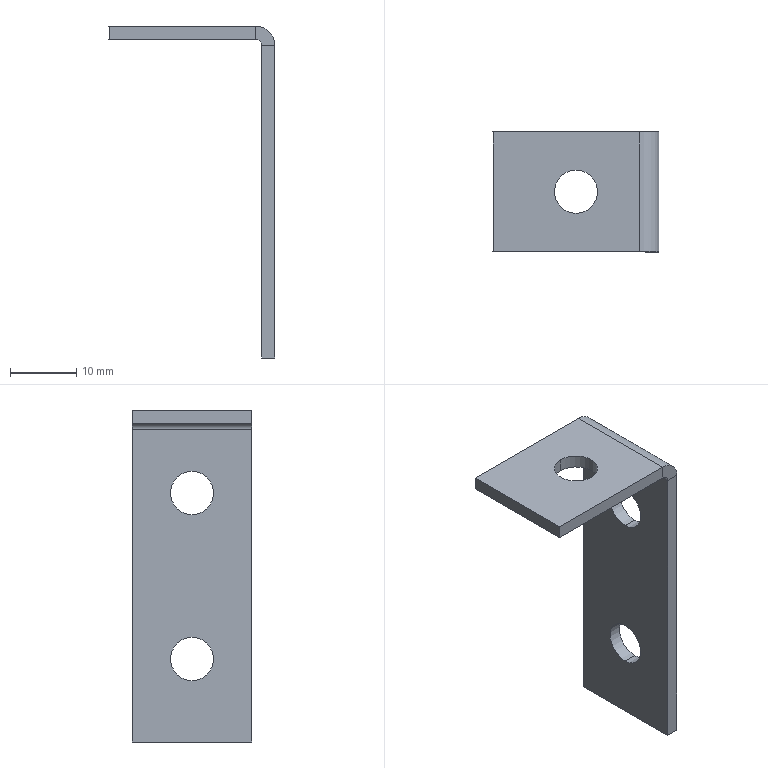Component | SolidWorks | Bracket(No.35)-1 | 1 solid | 20 faces | box 25 x 18 x 50 mm | volume 2398 mm3 | plane 12 | cylinder 8 | commonest cylinder face diameters 6.5 x6 2 x1 6 x1 | material Plain Carbon Steel
STEP:
#1=COLOUR_RGB('',0.7922,0.8196,0.9333);
#2=FILL_AREA_STYLE_COLOUR('',#1);
#3=FILL_AREA_STYLE('',(#2));
#4=SURFACE_STYLE_FILL_AREA(#3);
#5=SURFACE_SIDE_STYLE('',(#4));
#6=SURFACE_STYLE_USAGE(.BOTH.,#5);
#7=PRESENTATION_STYLE_ASSIGNMENT((#6));
#8=CARTESIAN_POINT('',(13.287,15.128,-2.047));
#9=VERTEX_POINT('',#8);
#10=CARTESIAN_POINT('',(13.287,15.384,-2.047));
#11=VERTEX_POINT('',#10);
#12=CARTESIAN_POINT('',(13.287,15.256,-2.047));
#13=DIRECTION('',(0.,-0.,1.));
#14=DIRECTION('',(0.,1.,0.));
#15=AXIS2_PLACEMENT_3D('',#12,#13,#14);
#16=CIRCLE('',#15,0.128);
#17=EDGE_CURVE('',#9,#11,#16,.T.);
#18=ORIENTED_EDGE('',*,*,#17,.F.);
#19=CARTESIAN_POINT('',(13.287,15.128,-1.969));
#20=VERTEX_POINT('',#19);
#21=CARTESIAN_POINT('',(13.287,15.128,-2.047));
#22=DIRECTION('',(0.,-0.,1.));
#23=VECTOR('',#22,39.37);
#24=LINE('',#21,#23);
#25=EDGE_CURVE('',#9,#20,#24,.T.);
#26=ORIENTED_EDGE('',*,*,#25,.T.);
#27=CARTESIAN_POINT('',(13.287,15.384,-1.969));
#28=VERTEX_POINT('',#27);
#29=CARTESIAN_POINT('',(13.287,15.256,-1.969));
#30=DIRECTION('',(0.,-0.,1.));
#31=DIRECTION('',(0.,1.,0.));
#32=AXIS2_PLACEMENT_3D('',#29,#30,#31);
#33=CIRCLE('',#32,0.128);
#34=EDGE_CURVE('',#20,#28,#33,.T.);
#35=ORIENTED_EDGE('',*,*,#34,.T.);
#36=CARTESIAN_POINT('',(13.287,15.384,-2.047));
#37=DIRECTION('',(0.,-0.,1.));
#38=VECTOR('',#37,39.37);
#39=LINE('',#36,#38);
#40=EDGE_CURVE('',#11,#28,#39,.T.);
#41=ORIENTED_EDGE('',*,*,#40,.F.);
#42=EDGE_LOOP('',(#18,#26,#35,#41));
#43=FACE_OUTER_BOUND('',#42,.T.);
#44=CARTESIAN_POINT('',(13.287,15.256,-2.047));
#45=DIRECTION('',(0.,-0.,1.));
#46=DIRECTION('',(0.,1.,0.));
#47=AXIS2_PLACEMENT_3D('',#44,#45,#46);
#48=CYLINDRICAL_SURFACE('',#47,0.128);
#49=ADVANCED_FACE('',(#43),#48,.F.);
#50=CARTESIAN_POINT('',(13.78,15.256,-2.333));
#51=VERTEX_POINT('',#50);
#52=CARTESIAN_POINT('',(13.78,15.256,-2.589));
#53=VERTEX_POINT('',#52);
#54=CARTESIAN_POINT('',(13.78,15.256,-2.461));
#55=DIRECTION('',(-1.,-0.,-0.));
#56=DIRECTION('',(0.,0.,-1.));
#57=AXIS2_PLACEMENT_3D('',#54,#55,#56);
#58=CIRCLE('',#57,0.128);
#59=EDGE_CURVE('',#51,#53,#58,.T.);
#60=ORIENTED_EDGE('',*,*,#59,.F.);
#61=CARTESIAN_POINT('',(13.701,15.256,-2.333));
#62=VERTEX_POINT('',#61);
#63=CARTESIAN_POINT('',(13.78,15.256,-2.333));
#64=DIRECTION('',(-1.,-0.,-0.));
#65=VECTOR('',#64,39.37);
#66=LINE('',#63,#65);
#67=EDGE_CURVE('',#51,#62,#66,.T.);
#68=ORIENTED_EDGE('',*,*,#67,.T.);
#69=CARTESIAN_POINT('',(13.701,15.256,-2.589));
#70=VERTEX_POINT('',#69);
#71=CARTESIAN_POINT('',(13.701,15.256,-2.461));
#72=DIRECTION('',(-1.,-0.,-0.));
#73=DIRECTION('',(0.,0.,-1.));
#74=AXIS2_PLACEMENT_3D('',#71,#72,#73);
#75=CIRCLE('',#74,0.128);
#76=EDGE_CURVE('',#62,#70,#75,.T.);
#77=ORIENTED_EDGE('',*,*,#76,.T.);
#78=CARTESIAN_POINT('',(13.78,15.256,-2.589));
#79=DIRECTION('',(-1.,-0.,-0.));
#80=VECTOR('',#79,39.37);
#81=LINE('',#78,#80);
#82=EDGE_CURVE('',#53,#70,#81,.T.);
#83=ORIENTED_EDGE('',*,*,#82,.F.);
#84=EDGE_LOOP('',(#60,#68,#77,#83));
#85=FACE_OUTER_BOUND('',#84,.T.);
#86=CARTESIAN_POINT('',(13.78,15.256,-2.461));
#87=DIRECTION('',(-1.,-0.,-0.));
#88=DIRECTION('',(0.,0.,-1.));
#89=AXIS2_PLACEMENT_3D('',#86,#87,#88);
#90=CYLINDRICAL_SURFACE('',#89,0.128);
#91=ADVANCED_FACE('',(#85),#90,.F.);
#92=CARTESIAN_POINT('',(13.78,15.256,-3.317));
#93=VERTEX_POINT('',#92);
#94=CARTESIAN_POINT('',(13.78,15.256,-3.573));
#95=VERTEX_POINT('',#94);
#96=CARTESIAN_POINT('',(13.78,15.256,-3.445));
#97=DIRECTION('',(-1.,-0.,-0.));
#98=DIRECTION('',(0.,0.,-1.));
#99=AXIS2_PLACEMENT_3D('',#96,#97,#98);
#100=CIRCLE('',#99,0.128);
#101=EDGE_CURVE('',#93,#95,#100,.T.);
#102=ORIENTED_EDGE('',*,*,#101,.F.);
#103=CARTESIAN_POINT('',(13.701,15.256,-3.317));
#104=VERTEX_POINT('',#103);
#105=CARTESIAN_POINT('',(13.78,15.256,-3.317));
#106=DIRECTION('',(-1.,-0.,-0.));
#107=VECTOR('',#106,39.37);
#108=LINE('',#105,#107);
#109=EDGE_CURVE('',#93,#104,#108,.T.);
#110=ORIENTED_EDGE('',*,*,#109,.T.);
#111=CARTESIAN_POINT('',(13.701,15.256,-3.573));
#112=VERTEX_POINT('',#111);
#113=CARTESIAN_POINT('',(13.701,15.256,-3.445));
#114=DIRECTION('',(-1.,-0.,-0.));
#115=DIRECTION('',(0.,0.,-1.));
#116=AXIS2_PLACEMENT_3D('',#113,#114,#115);
#117=CIRCLE('',#116,0.128);
#118=EDGE_CURVE('',#104,#112,#117,.T.);
#119=ORIENTED_EDGE('',*,*,#118,.T.);
#120=CARTESIAN_POINT('',(13.78,15.256,-3.573));
#121=DIRECTION('',(-1.,-0.,-0.));
#122=VECTOR('',#121,39.37);
#123=LINE('',#120,#122);
#124=EDGE_CURVE('',#95,#112,#123,.T.);
#125=ORIENTED_EDGE('',*,*,#124,.F.);
#126=EDGE_LOOP('',(#102,#110,#119,#125));
#127=FACE_OUTER_BOUND('',#126,.T.);
#128=CARTESIAN_POINT('',(13.78,15.256,-3.445));
#129=DIRECTION('',(-1.,-0.,-0.));
#130=DIRECTION('',(0.,0.,-1.));
#131=AXIS2_PLACEMENT_3D('',#128,#129,#130);
#132=CYLINDRICAL_SURFACE('',#131,0.128);
#133=ADVANCED_FACE('',(#127),#132,.F.);
#134=CARTESIAN_POINT('',(13.78,14.902,-2.087));
#135=VERTEX_POINT('',#134);
#136=CARTESIAN_POINT('',(13.701,14.902,-2.087));
#137=VERTEX_POINT('',#136);
#138=CARTESIAN_POINT('',(13.78,14.902,-2.087));
#139=DIRECTION('',(-1.,-0.,0.));
#140=VECTOR('',#139,39.37);
#141=LINE('',#138,#140);
#142=EDGE_CURVE('',#135,#137,#141,.T.);
#143=ORIENTED_EDGE('',*,*,#142,.F.);
#144=CARTESIAN_POINT('',(13.661,14.902,-1.969));
#145=VERTEX_POINT('',#144);
#146=CARTESIAN_POINT('',(13.661,14.902,-2.087));
#147=DIRECTION('',(0.,-1.,-0.));
#148=DIRECTION('',(1.,0.,0.));
#149=AXIS2_PLACEMENT_3D('',#146,#147,#148);
#150=CIRCLE('',#149,0.1181);
#151=EDGE_CURVE('',#135,#145,#150,.T.);
#152=ORIENTED_EDGE('',*,*,#151,.T.);
#153=CARTESIAN_POINT('',(13.661,14.902,-2.047));
#154=VERTEX_POINT('',#153);
#155=CARTESIAN_POINT('',(13.661,14.902,-2.047));
#156=DIRECTION('',(0.,-0.,1.));
#157=VECTOR('',#156,39.37);
#158=LINE('',#155,#157);
#159=EDGE_CURVE('',#154,#145,#158,.T.);
#160=ORIENTED_EDGE('',*,*,#159,.F.);
#161=CARTESIAN_POINT('',(13.661,14.902,-2.087));
#162=DIRECTION('',(0.,-1.,-0.));
#163=DIRECTION('',(-1.,0.,0.));
#164=AXIS2_PLACEMENT_3D('',#161,#162,#163);
#165=CIRCLE('',#164,0.03937);
#166=EDGE_CURVE('',#137,#154,#165,.T.);
#167=ORIENTED_EDGE('',*,*,#166,.F.);
#168=EDGE_LOOP('',(#143,#152,#160,#167));
#169=FACE_OUTER_BOUND('',#168,.T.);
#170=CARTESIAN_POINT('',(13.78,14.902,-2.087));
#171=DIRECTION('',(0.,-1.,-0.));
#172=DIRECTION('',(-1.,-0.,0.));
#173=AXIS2_PLACEMENT_3D('',#170,#171,#172);
#174=PLANE('',#173);
#175=ADVANCED_FACE('',(#169),#174,.T.);
#176=CARTESIAN_POINT('',(13.78,14.902,-3.937));
#177=VERTEX_POINT('',#176);
#178=CARTESIAN_POINT('',(13.78,14.902,-3.937));
#179=DIRECTION('',(-0.,-0.,1.));
#180=VECTOR('',#179,39.37);
#181=LINE('',#178,#180);
#182=EDGE_CURVE('',#177,#135,#181,.T.);
#183=ORIENTED_EDGE('',*,*,#182,.T.);
#184=ORIENTED_EDGE('',*,*,#142,.T.);
#185=CARTESIAN_POINT('',(13.701,14.902,-3.937));
#186=VERTEX_POINT('',#185);
#187=CARTESIAN_POINT('',(13.701,14.902,-3.937));
#188=DIRECTION('',(-0.,-0.,1.));
#189=VECTOR('',#188,39.37);
#190=LINE('',#187,#189);
#191=EDGE_CURVE('',#186,#137,#190,.T.);
#192=ORIENTED_EDGE('',*,*,#191,.F.);
#193=CARTESIAN_POINT('',(13.78,14.902,-3.937));
#194=DIRECTION('',(-1.,-0.,0.));
#195=VECTOR('',#194,39.37);
#196=LINE('',#193,#195);
#197=EDGE_CURVE('',#177,#186,#196,.T.);
#198=ORIENTED_EDGE('',*,*,#197,.F.);
#199=EDGE_LOOP('',(#183,#184,#192,#198));
#200=FACE_OUTER_BOUND('',#199,.T.);
#201=CARTESIAN_POINT('',(13.661,14.902,-2.047));
#202=DIRECTION('',(0.,-1.,-0.));
#203=DIRECTION('',(-1.,-0.,0.));
#204=AXIS2_PLACEMENT_3D('',#201,#202,#203);
#205=PLANE('',#204);
#206=ADVANCED_FACE('',(#200),#205,.T.);
#207=CARTESIAN_POINT('',(13.661,15.61,-1.969));
#208=VERTEX_POINT('',#207);
#209=CARTESIAN_POINT('',(13.661,15.61,-2.047));
#210=VERTEX_POINT('',#209);
#211=CARTESIAN_POINT('',(13.661,15.61,-1.969));
#212=DIRECTION('',(-0.,0.,-1.));
#213=VECTOR('',#212,39.37);
#214=LINE('',#211,#213);
#215=EDGE_CURVE('',#208,#210,#214,.T.);
#216=ORIENTED_EDGE('',*,*,#215,.F.);
#217=CARTESIAN_POINT('',(13.78,15.61,-2.087));
#218=VERTEX_POINT('',#217);
#219=CARTESIAN_POINT('',(13.661,15.61,-2.087));
#220=DIRECTION('',(0.,-1.,-0.));
#221=DIRECTION('',(1.,0.,0.));
#222=AXIS2_PLACEMENT_3D('',#219,#220,#221);
#223=CIRCLE('',#222,0.1181);
#224=EDGE_CURVE('',#218,#208,#223,.T.);
#225=ORIENTED_EDGE('',*,*,#224,.F.);
#226=CARTESIAN_POINT('',(13.701,15.61,-2.087));
#227=VERTEX_POINT('',#226);
#228=CARTESIAN_POINT('',(13.701,15.61,-2.087));
#229=DIRECTION('',(1.,0.,-0.));
#230=VECTOR('',#229,39.37);
#231=LINE('',#228,#230);
#232=EDGE_CURVE('',#227,#218,#231,.T.);
#233=ORIENTED_EDGE('',*,*,#232,.F.);
#234=CARTESIAN_POINT('',(13.661,15.61,-2.087));
#235=DIRECTION('',(0.,-1.,-0.));
#236=DIRECTION('',(-1.,0.,0.));
#237=AXIS2_PLACEMENT_3D('',#234,#235,#236);
#238=CIRCLE('',#237,0.03937);
#239=EDGE_CURVE('',#227,#210,#238,.T.);
#240=ORIENTED_EDGE('',*,*,#239,.T.);
#241=EDGE_LOOP('',(#216,#225,#233,#240));
#242=FACE_OUTER_BOUND('',#241,.T.);
#243=CARTESIAN_POINT('',(13.661,15.61,-1.969));
#244=DIRECTION('',(-0.,1.,0.));
#245=DIRECTION('',(1.,0.,-0.));
#246=AXIS2_PLACEMENT_3D('',#243,#244,#245);
#247=PLANE('',#246);
#248=ADVANCED_FACE('',(#242),#247,.T.);
#249=CARTESIAN_POINT('',(12.795,15.61,-1.969));
#250=VERTEX_POINT('',#249);
#251=CARTESIAN_POINT('',(13.78,15.61,-1.969));
#252=DIRECTION('',(-1.,-0.,0.));
#253=VECTOR('',#252,39.37);
#254=LINE('',#251,#253);
#255=EDGE_CURVE('',#208,#250,#254,.T.);
#256=ORIENTED_EDGE('',*,*,#255,.F.);
#257=ORIENTED_EDGE('',*,*,#215,.T.);
#258=CARTESIAN_POINT('',(12.795,15.61,-2.047));
#259=VERTEX_POINT('',#258);
#260=CARTESIAN_POINT('',(13.78,15.61,-2.047));
#261=DIRECTION('',(-1.,-0.,0.));
#262=VECTOR('',#261,39.37);
#263=LINE('',#260,#262);
#264=EDGE_CURVE('',#210,#259,#263,.T.);
#265=ORIENTED_EDGE('',*,*,#264,.T.);
#266=CARTESIAN_POINT('',(12.795,15.61,-2.047));
#267=DIRECTION('',(0.,-0.,1.));
#268=VECTOR('',#267,39.37);
#269=LINE('',#266,#268);
#270=EDGE_CURVE('',#259,#250,#269,.T.);
#271=ORIENTED_EDGE('',*,*,#270,.T.);
#272=EDGE_LOOP('',(#256,#257,#265,#271));
#273=FACE_OUTER_BOUND('',#272,.T.);
#274=CARTESIAN_POINT('',(13.701,15.61,-2.087));
#275=DIRECTION('',(-0.,1.,0.));
#276=DIRECTION('',(1.,0.,-0.));
#277=AXIS2_PLACEMENT_3D('',#274,#275,#276);
#278=PLANE('',#277);
#279=ADVANCED_FACE('',(#273),#278,.T.);
#280=CARTESIAN_POINT('',(13.287,15.256,-1.969));
#281=DIRECTION('',(0.,-0.,1.));
#282=DIRECTION('',(0.,1.,0.));
#283=AXIS2_PLACEMENT_3D('',#280,#281,#282);
#284=CIRCLE('',#283,0.128);
#285=EDGE_CURVE('',#28,#20,#284,.T.);
#286=ORIENTED_EDGE('',*,*,#285,.F.);
#287=ORIENTED_EDGE('',*,*,#34,.F.);
#288=EDGE_LOOP('',(#286,#287));
#289=FACE_BOUND('',#288,.T.);
#290=ORIENTED_EDGE('',*,*,#255,.T.);
#291=CARTESIAN_POINT('',(12.795,14.902,-1.969));
#292=VERTEX_POINT('',#291);
#293=CARTESIAN_POINT('',(12.795,14.902,-1.969));
#294=DIRECTION('',(-0.,1.,0.));
#295=VECTOR('',#294,39.37);
#296=LINE('',#293,#295);
#297=EDGE_CURVE('',#292,#250,#296,.T.);
#298=ORIENTED_EDGE('',*,*,#297,.F.);
#299=CARTESIAN_POINT('',(13.78,14.902,-1.969));
#300=DIRECTION('',(-1.,-0.,0.));
#301=VECTOR('',#300,39.37);
#302=LINE('',#299,#301);
#303=EDGE_CURVE('',#145,#292,#302,.T.);
#304=ORIENTED_EDGE('',*,*,#303,.F.);
#305=CARTESIAN_POINT('',(13.661,14.902,-1.969));
#306=DIRECTION('',(-0.,1.,0.));
#307=VECTOR('',#306,39.37);
#308=LINE('',#305,#307);
#309=EDGE_CURVE('',#145,#208,#308,.T.);
#310=ORIENTED_EDGE('',*,*,#309,.T.);
#311=EDGE_LOOP('',(#290,#298,#304,#310));
#312=FACE_OUTER_BOUND('',#311,.T.);
#313=CARTESIAN_POINT('',(13.78,14.902,-1.969));
#314=DIRECTION('',(-0.,0.,-1.));
#315=DIRECTION('',(0.,-1.,-0.));
#316=AXIS2_PLACEMENT_3D('',#313,#314,#315);
#317=PLANE('',#316);
#318=ADVANCED_FACE('',(#289,#312),#317,.F.);
#319=ORIENTED_EDGE('',*,*,#270,.F.);
#320=CARTESIAN_POINT('',(12.795,14.902,-2.047));
#321=VERTEX_POINT('',#320);
#322=CARTESIAN_POINT('',(12.795,14.902,-2.047));
#323=DIRECTION('',(-0.,1.,0.));
#324=VECTOR('',#323,39.37);
#325=LINE('',#322,#324);
#326=EDGE_CURVE('',#321,#259,#325,.T.);
#327=ORIENTED_EDGE('',*,*,#326,.F.);
#328=CARTESIAN_POINT('',(12.795,14.902,-2.047));
#329=DIRECTION('',(0.,-0.,1.));
#330=VECTOR('',#329,39.37);
#331=LINE('',#328,#330);
#332=EDGE_CURVE('',#321,#292,#331,.T.);
#333=ORIENTED_EDGE('',*,*,#332,.T.);
#334=ORIENTED_EDGE('',*,*,#297,.T.);
#335=EDGE_LOOP('',(#319,#327,#333,#334));
#336=FACE_OUTER_BOUND('',#335,.T.);
#337=CARTESIAN_POINT('',(12.795,14.902,-2.047));
#338=DIRECTION('',(-1.,-0.,0.));
#339=DIRECTION('',(-0.,1.,0.));
#340=AXIS2_PLACEMENT_3D('',#337,#338,#339);
#341=PLANE('',#340);
#342=ADVANCED_FACE('',(#336),#341,.T.);
#343=CARTESIAN_POINT('',(13.287,15.256,-2.047));
#344=DIRECTION('',(0.,-0.,1.));
#345=DIRECTION('',(0.,1.,0.));
#346=AXIS2_PLACEMENT_3D('',#343,#344,#345);
#347=CIRCLE('',#346,0.128);
#348=EDGE_CURVE('',#11,#9,#347,.T.);
#349=ORIENTED_EDGE('',*,*,#348,.T.);
#350=ORIENTED_EDGE('',*,*,#17,.T.);
#351=EDGE_LOOP('',(#349,#350));
#352=FACE_BOUND('',#351,.T.);
#353=ORIENTED_EDGE('',*,*,#264,.F.);
#354=CARTESIAN_POINT('',(13.661,14.902,-2.047));
#355=DIRECTION('',(-0.,1.,0.));
#356=VECTOR('',#355,39.37);
#357=LINE('',#354,#356);
#358=EDGE_CURVE('',#154,#210,#357,.T.);
#359=ORIENTED_EDGE('',*,*,#358,.F.);
#360=CARTESIAN_POINT('',(13.78,14.902,-2.047));
#361=DIRECTION('',(-1.,-0.,0.));
#362=VECTOR('',#361,39.37);
#363=LINE('',#360,#362);
#364=EDGE_CURVE('',#154,#321,#363,.T.);
#365=ORIENTED_EDGE('',*,*,#364,.T.);
#366=ORIENTED_EDGE('',*,*,#326,.T.);
#367=EDGE_LOOP('',(#353,#359,#365,#366));
#368=FACE_OUTER_BOUND('',#367,.T.);
#369=CARTESIAN_POINT('',(13.78,14.902,-2.047));
#370=DIRECTION('',(-0.,0.,-1.));
#371=DIRECTION('',(0.,-1.,-0.));
#372=AXIS2_PLACEMENT_3D('',#369,#370,#371);
#373=PLANE('',#372);
#374=ADVANCED_FACE('',(#352,#368),#373,.T.);
#375=ORIENTED_EDGE('',*,*,#239,.F.);
#376=CARTESIAN_POINT('',(13.701,14.902,-2.087));
#377=DIRECTION('',(-0.,1.,0.));
#378=VECTOR('',#377,39.37);
#379=LINE('',#376,#378);
#380=EDGE_CURVE('',#137,#227,#379,.T.);
#381=ORIENTED_EDGE('',*,*,#380,.F.);
#382=ORIENTED_EDGE('',*,*,#166,.T.);
#383=ORIENTED_EDGE('',*,*,#358,.T.);
#384=EDGE_LOOP('',(#375,#381,#382,#383));
#385=FACE_OUTER_BOUND('',#384,.T.);
#386=CARTESIAN_POINT('',(13.661,14.902,-2.087));
#387=DIRECTION('',(-0.,1.,0.));
#388=DIRECTION('',(1.,0.,0.));
#389=AXIS2_PLACEMENT_3D('',#386,#387,#388);
#390=CYLINDRICAL_SURFACE('',#389,0.03937);
#391=ADVANCED_FACE('',(#385),#390,.F.);
#392=CARTESIAN_POINT('',(13.701,15.256,-2.461));
#393=DIRECTION('',(-1.,-0.,-0.));
#394=DIRECTION('',(0.,0.,-1.));
#395=AXIS2_PLACEMENT_3D('',#392,#393,#394);
#396=CIRCLE('',#395,0.128);
#397=EDGE_CURVE('',#70,#62,#396,.T.);
#398=ORIENTED_EDGE('',*,*,#397,.F.);
#399=ORIENTED_EDGE('',*,*,#76,.F.);
#400=EDGE_LOOP('',(#398,#399));
#401=FACE_BOUND('',#400,.T.);
#402=CARTESIAN_POINT('',(13.701,15.256,-3.445));
#403=DIRECTION('',(-1.,-0.,-0.));
#404=DIRECTION('',(0.,0.,-1.));
#405=AXIS2_PLACEMENT_3D('',#402,#403,#404);
#406=CIRCLE('',#405,0.128);
#407=EDGE_CURVE('',#112,#104,#406,.T.);
#408=ORIENTED_EDGE('',*,*,#407,.F.);
#409=ORIENTED_EDGE('',*,*,#118,.F.);
#410=EDGE_LOOP('',(#408,#409));
#411=FACE_BOUND('',#410,.T.);
#412=CARTESIAN_POINT('',(13.701,15.61,-3.937));
#413=VERTEX_POINT('',#412);
#414=CARTESIAN_POINT('',(13.701,15.61,-3.937));
#415=DIRECTION('',(-0.,-0.,1.));
#416=VECTOR('',#415,39.37);
#417=LINE('',#414,#416);
#418=EDGE_CURVE('',#413,#227,#417,.T.);
#419=ORIENTED_EDGE('',*,*,#418,.F.);
#420=CARTESIAN_POINT('',(13.701,14.902,-3.937));
#421=DIRECTION('',(-0.,1.,0.));
#422=VECTOR('',#421,39.37);
#423=LINE('',#420,#422);
#424=EDGE_CURVE('',#186,#413,#423,.T.);
#425=ORIENTED_EDGE('',*,*,#424,.F.);
#426=ORIENTED_EDGE('',*,*,#191,.T.);
#427=ORIENTED_EDGE('',*,*,#380,.T.);
#428=EDGE_LOOP('',(#419,#425,#426,#427));
#429=FACE_OUTER_BOUND('',#428,.T.);
#430=CARTESIAN_POINT('',(13.701,14.902,-3.937));
#431=DIRECTION('',(-1.,-0.,-0.));
#432=DIRECTION('',(0.,0.,-1.));
#433=AXIS2_PLACEMENT_3D('',#430,#431,#432);
#434=PLANE('',#433);
#435=ADVANCED_FACE('',(#401,#411,#429),#434,.T.);
#436=CARTESIAN_POINT('',(13.78,15.61,-3.937));
#437=VERTEX_POINT('',#436);
#438=CARTESIAN_POINT('',(13.78,15.61,-3.937));
#439=DIRECTION('',(-1.,-0.,0.));
#440=VECTOR('',#439,39.37);
#441=LINE('',#438,#440);
#442=EDGE_CURVE('',#437,#413,#441,.T.);
#443=ORIENTED_EDGE('',*,*,#442,.F.);
#444=CARTESIAN_POINT('',(13.78,14.902,-3.937));
#445=DIRECTION('',(-0.,1.,0.));
#446=VECTOR('',#445,39.37);
#447=LINE('',#444,#446);
#448=EDGE_CURVE('',#177,#437,#447,.T.);
#449=ORIENTED_EDGE('',*,*,#448,.F.);
#450=ORIENTED_EDGE('',*,*,#197,.T.);
#451=ORIENTED_EDGE('',*,*,#424,.T.);
#452=EDGE_LOOP('',(#443,#449,#450,#451));
#453=FACE_OUTER_BOUND('',#452,.T.);
#454=CARTESIAN_POINT('',(13.78,14.902,-3.937));
#455=DIRECTION('',(-0.,0.,-1.));
#456=DIRECTION('',(0.,-1.,-0.));
#457=AXIS2_PLACEMENT_3D('',#454,#455,#456);
#458=PLANE('',#457);
#459=ADVANCED_FACE('',(#453),#458,.T.);
#460=CARTESIAN_POINT('',(13.78,15.256,-2.461));
#461=DIRECTION('',(-1.,-0.,-0.));
#462=DIRECTION('',(0.,0.,-1.));
#463=AXIS2_PLACEMENT_3D('',#460,#461,#462);
#464=CIRCLE('',#463,0.128);
#465=EDGE_CURVE('',#53,#51,#464,.T.);
#466=ORIENTED_EDGE('',*,*,#465,.T.);
#467=ORIENTED_EDGE('',*,*,#59,.T.);
#468=EDGE_LOOP('',(#466,#467));
#469=FACE_BOUND('',#468,.T.);
#470=CARTESIAN_POINT('',(13.78,15.256,-3.445));
#471=DIRECTION('',(-1.,-0.,-0.));
#472=DIRECTION('',(0.,0.,-1.));
#473=AXIS2_PLACEMENT_3D('',#470,#471,#472);
#474=CIRCLE('',#473,0.128);
#475=EDGE_CURVE('',#95,#93,#474,.T.);
#476=ORIENTED_EDGE('',*,*,#475,.T.);
#477=ORIENTED_EDGE('',*,*,#101,.T.);
#478=EDGE_LOOP('',(#476,#477));
#479=FACE_BOUND('',#478,.T.);
#480=CARTESIAN_POINT('',(13.78,15.61,-3.937));
#481=DIRECTION('',(-0.,-0.,1.));
#482=VECTOR('',#481,39.37);
#483=LINE('',#480,#482);
#484=EDGE_CURVE('',#437,#218,#483,.T.);
#485=ORIENTED_EDGE('',*,*,#484,.T.);
#486=CARTESIAN_POINT('',(13.78,14.902,-2.087));
#487=DIRECTION('',(-0.,1.,0.));
#488=VECTOR('',#487,39.37);
#489=LINE('',#486,#488);
#490=EDGE_CURVE('',#135,#218,#489,.T.);
#491=ORIENTED_EDGE('',*,*,#490,.F.);
#492=ORIENTED_EDGE('',*,*,#182,.F.);
#493=ORIENTED_EDGE('',*,*,#448,.T.);
#494=EDGE_LOOP('',(#485,#491,#492,#493));
#495=FACE_OUTER_BOUND('',#494,.T.);
#496=CARTESIAN_POINT('',(13.78,14.902,-3.937));
#497=DIRECTION('',(-1.,-0.,-0.));
#498=DIRECTION('',(0.,0.,-1.));
#499=AXIS2_PLACEMENT_3D('',#496,#497,#498);
#500=PLANE('',#499);
#501=ADVANCED_FACE('',(#469,#479,#495),#500,.F.);
#502=ORIENTED_EDGE('',*,*,#224,.T.);
#503=ORIENTED_EDGE('',*,*,#309,.F.);
#504=ORIENTED_EDGE('',*,*,#151,.F.);
#505=ORIENTED_EDGE('',*,*,#490,.T.);
#506=EDGE_LOOP('',(#502,#503,#504,#505));
#507=FACE_OUTER_BOUND('',#506,.T.);
#508=CARTESIAN_POINT('',(13.661,14.902,-2.087));
#509=DIRECTION('',(-0.,1.,0.));
#510=DIRECTION('',(1.,0.,0.));
#511=AXIS2_PLACEMENT_3D('',#508,#509,#510);
#512=CYLINDRICAL_SURFACE('',#511,0.1181);
#513=ADVANCED_FACE('',(#507),#512,.T.);
#514=ORIENTED_EDGE('',*,*,#303,.T.);
#515=ORIENTED_EDGE('',*,*,#332,.F.);
#516=ORIENTED_EDGE('',*,*,#364,.F.);
#517=ORIENTED_EDGE('',*,*,#159,.T.);
#518=EDGE_LOOP('',(#514,#515,#516,#517));
#519=FACE_OUTER_BOUND('',#518,.T.);
#520=CARTESIAN_POINT('',(13.661,14.902,-2.087));
#521=DIRECTION('',(0.,-1.,-0.));
#522=DIRECTION('',(-1.,-0.,0.));
#523=AXIS2_PLACEMENT_3D('',#520,#521,#522);
#524=PLANE('',#523);
#525=ADVANCED_FACE('',(#519),#524,.T.);
#526=ORIENTED_EDGE('',*,*,#418,.T.);
#527=ORIENTED_EDGE('',*,*,#232,.T.);
#528=ORIENTED_EDGE('',*,*,#484,.F.);
#529=ORIENTED_EDGE('',*,*,#442,.T.);
#530=EDGE_LOOP('',(#526,#527,#528,#529));
#531=FACE_OUTER_BOUND('',#530,.T.);
#532=CARTESIAN_POINT('',(13.661,15.61,-2.087));
#533=DIRECTION('',(0.,-1.,-0.));
#534=DIRECTION('',(-1.,-0.,0.));
#535=AXIS2_PLACEMENT_3D('',#532,#533,#534);
#536=PLANE('',#535);
#537=ADVANCED_FACE('',(#531),#536,.F.);
#538=ORIENTED_EDGE('',*,*,#109,.F.);
#539=ORIENTED_EDGE('',*,*,#475,.F.);
#540=ORIENTED_EDGE('',*,*,#124,.T.);
#541=ORIENTED_EDGE('',*,*,#407,.T.);
#542=EDGE_LOOP('',(#538,#539,#540,#541));
#543=FACE_OUTER_BOUND('',#542,.T.);
#544=CARTESIAN_POINT('',(13.78,15.256,-3.445));
#545=DIRECTION('',(-1.,-0.,-0.));
#546=DIRECTION('',(0.,0.,-1.));
#547=AXIS2_PLACEMENT_3D('',#544,#545,#546);
#548=CYLINDRICAL_SURFACE('',#547,0.128);
#549=ADVANCED_FACE('',(#543),#548,.F.);
#550=ORIENTED_EDGE('',*,*,#67,.F.);
#551=ORIENTED_EDGE('',*,*,#465,.F.);
#552=ORIENTED_EDGE('',*,*,#82,.T.);
#553=ORIENTED_EDGE('',*,*,#397,.T.);
#554=EDGE_LOOP('',(#550,#551,#552,#553));
#555=FACE_OUTER_BOUND('',#554,.T.);
#556=CARTESIAN_POINT('',(13.78,15.256,-2.461));
#557=DIRECTION('',(-1.,-0.,-0.));
#558=DIRECTION('',(0.,0.,-1.));
#559=AXIS2_PLACEMENT_3D('',#556,#557,#558);
#560=CYLINDRICAL_SURFACE('',#559,0.128);
#561=ADVANCED_FACE('',(#555),#560,.F.);
#562=ORIENTED_EDGE('',*,*,#25,.F.);
#563=ORIENTED_EDGE('',*,*,#348,.F.);
#564=ORIENTED_EDGE('',*,*,#40,.T.);
#565=ORIENTED_EDGE('',*,*,#285,.T.);
#566=EDGE_LOOP('',(#562,#563,#564,#565));
#567=FACE_OUTER_BOUND('',#566,.T.);
#568=CARTESIAN_POINT('',(13.287,15.256,-2.047));
#569=DIRECTION('',(0.,-0.,1.));
#570=DIRECTION('',(0.,1.,0.));
#571=AXIS2_PLACEMENT_3D('',#568,#569,#570);
#572=CYLINDRICAL_SURFACE('',#571,0.128);
#573=ADVANCED_FACE('',(#567),#572,.F.);
#574=CLOSED_SHELL('',(#49,#91,#133,#175,#206,#248,#279,#318,#342,#374,#391,#435,#459,#501,#513,#525,#537,#549,#561,#573));
#575=MANIFOLD_SOLID_BREP('',#574);
#576=STYLED_ITEM('',(#7),#575);
#577=(LENGTH_UNIT()NAMED_UNIT(*)SI_UNIT($,.METRE.));
#578=LENGTH_MEASURE_WITH_UNIT(LENGTH_MEASURE(0.0254),#577);
#579=DIMENSIONAL_EXPONENTS(1.,0.,0.,0.,0.,0.,0.);
#580=(CONVERSION_BASED_UNIT('',#578)LENGTH_UNIT()NAMED_UNIT(#579));
#581=UNCERTAINTY_MEASURE_WITH_UNIT(LENGTH_MEASURE(0.00001),#580,'','');
#582=(NAMED_UNIT(*)PLANE_ANGLE_UNIT()SI_UNIT($,.RADIAN.));
#583=(NAMED_UNIT(*)SI_UNIT($,.STERADIAN.)SOLID_ANGLE_UNIT());
#584=(GEOMETRIC_REPRESENTATION_CONTEXT(3)GLOBAL_UNCERTAINTY_ASSIGNED_CONTEXT((#581))GLOBAL_UNIT_ASSIGNED_CONTEXT((#580,#582,#583))REPRESENTATION_CONTEXT('',''));
#585=MECHANICAL_DESIGN_GEOMETRIC_PRESENTATION_REPRESENTATION('',(#576),#584);
#586=PRESENTATION_LAYER_ASSIGNMENT('','',(#576));
#587=CARTESIAN_POINT('',(0.,0.,0.));
#588=DIRECTION('',(0.,0.,1.));
#589=DIRECTION('',(1.,0.,0.));
#590=AXIS2_PLACEMENT_3D('',#587,#588,#589);
#591=(LENGTH_UNIT()NAMED_UNIT(*)SI_UNIT($,.METRE.));
#592=LENGTH_MEASURE_WITH_UNIT(LENGTH_MEASURE(0.0254),#591);
#593=DIMENSIONAL_EXPONENTS(1.,0.,0.,0.,0.,0.,0.);
#594=(CONVERSION_BASED_UNIT('',#592)LENGTH_UNIT()NAMED_UNIT(#593));
#595=UNCERTAINTY_MEASURE_WITH_UNIT(LENGTH_MEASURE(0.00001),#594,'','');
#596=(NAMED_UNIT(*)PLANE_ANGLE_UNIT()SI_UNIT($,.RADIAN.));
#597=(NAMED_UNIT(*)SI_UNIT($,.STERADIAN.)SOLID_ANGLE_UNIT());
#598=(GEOMETRIC_REPRESENTATION_CONTEXT(3)GLOBAL_UNCERTAINTY_ASSIGNED_CONTEXT((#595))GLOBAL_UNIT_ASSIGNED_CONTEXT((#594,#596,#597))REPRESENTATION_CONTEXT('',''));
#599=ADVANCED_BREP_SHAPE_REPRESENTATION('',(#575,#590),#598);